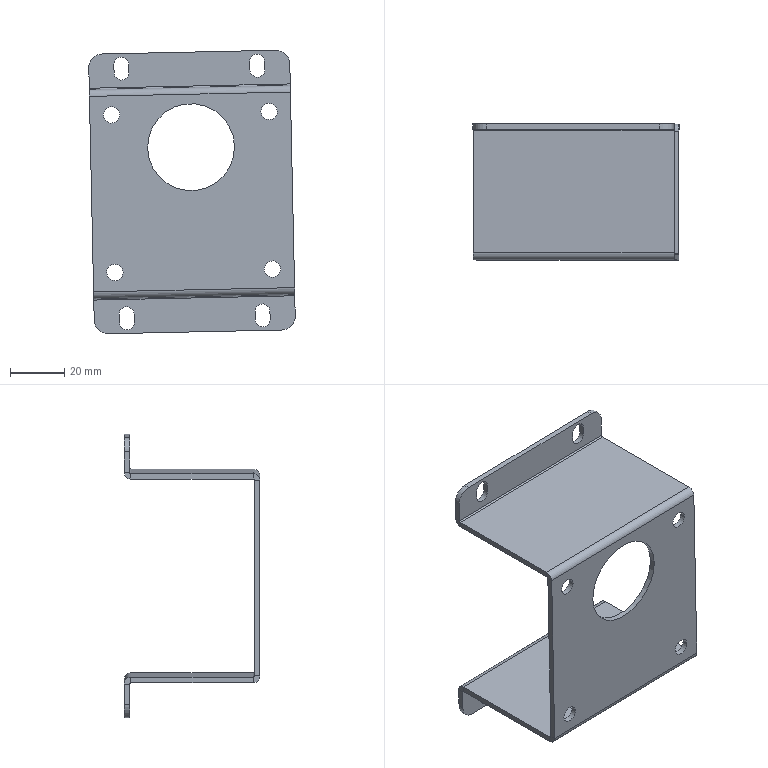Component | SolidWorks | MotorBracket-1 | 1 solid | 68 faces | volume 26871 mm3 | plane 38 | cylinder 30 | commonest cylinder face diameters 6 x8 5.5 x8 5 x4 1 x4 10 x4 32 x2